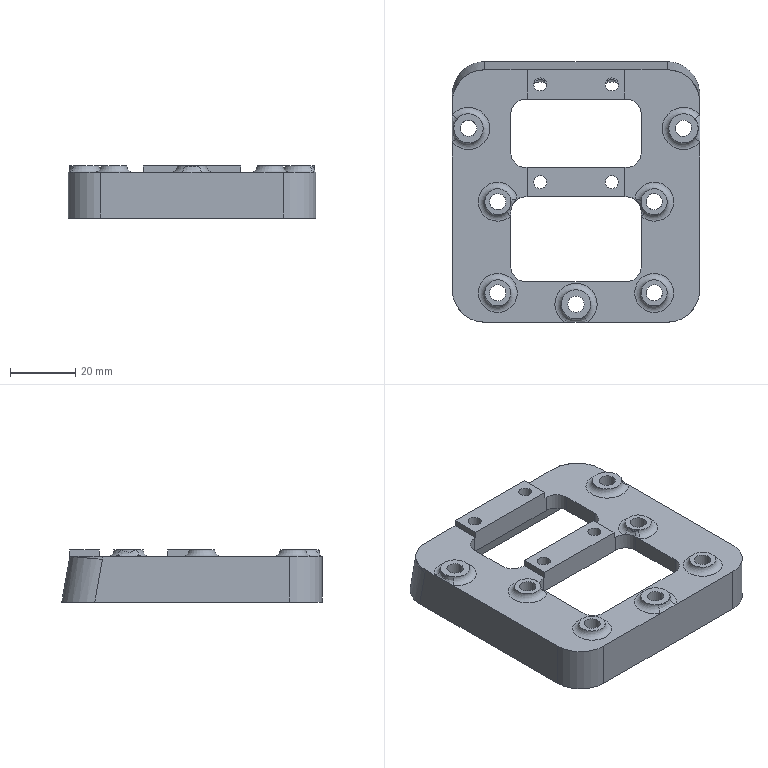Component | NX | BASE | 1 solid | 87 faces | volume 35871 mm3 | plane 39 | cylinder 32 | torus 7 | spline 7 | cone 2 | commonest cylinder face diameters 9 x11 5 x7 20 x6 4.024 x4 8 x2 3.3 x2